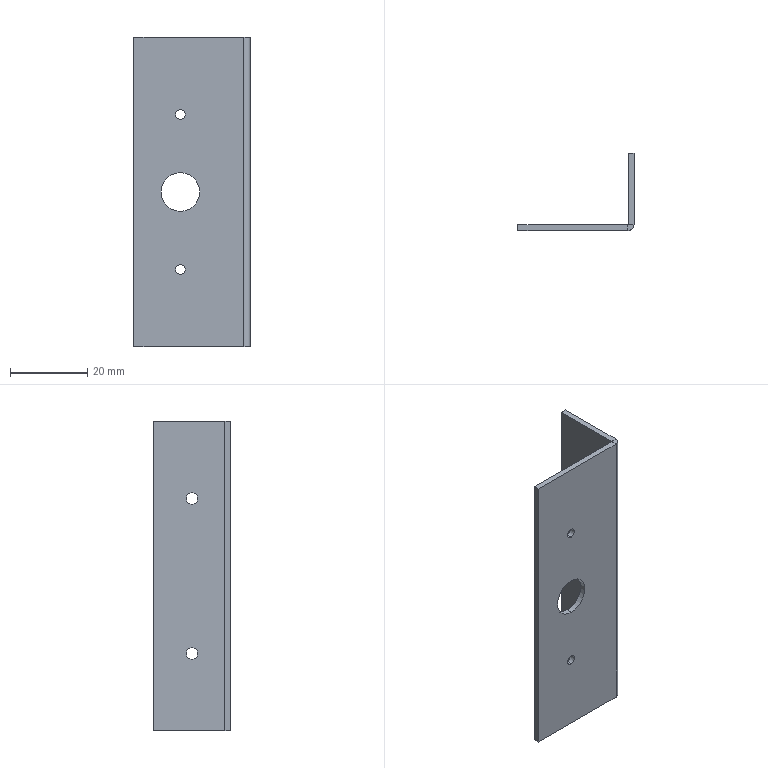Component | SolidWorks | LightBox-1_LampHolderMountingPlate-2 | 1 solid | 24 faces | box 30 x 20 x 80 mm | volume 5622 mm3 | cylinder 12 | plane 12 | commonest cylinder face diameters 3 x4 2.5 x4 10 x2 3.2 x1 0.2 x1
STEP:
#1=COLOUR_RGB('',0.7922,0.8196,0.9333);
#2=FILL_AREA_STYLE_COLOUR('',#1);
#3=FILL_AREA_STYLE('',(#2));
#4=SURFACE_STYLE_FILL_AREA(#3);
#5=SURFACE_SIDE_STYLE('',(#4));
#6=SURFACE_STYLE_USAGE(.BOTH.,#5);
#7=PRESENTATION_STYLE_ASSIGNMENT((#6));
#8=CARTESIAN_POINT('',(4.946,-0.2593,2.362));
#9=VERTEX_POINT('',#8);
#10=CARTESIAN_POINT('',(4.946,-0.1412,2.362));
#11=VERTEX_POINT('',#10);
#12=CARTESIAN_POINT('',(4.946,-0.2003,2.362));
#13=DIRECTION('',(1.,-0.,0.));
#14=DIRECTION('',(0.,1.,0.));
#15=AXIS2_PLACEMENT_3D('',#12,#13,#14);
#16=CIRCLE('',#15,0.05906);
#17=EDGE_CURVE('',#9,#11,#16,.T.);
#18=ORIENTED_EDGE('',*,*,#17,.F.);
#19=CARTESIAN_POINT('',(5.006,-0.2593,2.362));
#20=VERTEX_POINT('',#19);
#21=CARTESIAN_POINT('',(4.946,-0.2593,2.362));
#22=DIRECTION('',(1.,-0.,0.));
#23=VECTOR('',#22,39.37);
#24=LINE('',#21,#23);
#25=EDGE_CURVE('',#9,#20,#24,.T.);
#26=ORIENTED_EDGE('',*,*,#25,.T.);
#27=CARTESIAN_POINT('',(5.006,-0.1412,2.362));
#28=VERTEX_POINT('',#27);
#29=CARTESIAN_POINT('',(5.006,-0.2003,2.362));
#30=DIRECTION('',(1.,-0.,0.));
#31=DIRECTION('',(0.,1.,0.));
#32=AXIS2_PLACEMENT_3D('',#29,#30,#31);
#33=CIRCLE('',#32,0.05906);
#34=EDGE_CURVE('',#20,#28,#33,.T.);
#35=ORIENTED_EDGE('',*,*,#34,.T.);
#36=CARTESIAN_POINT('',(4.946,-0.1412,2.362));
#37=DIRECTION('',(1.,-0.,0.));
#38=VECTOR('',#37,39.37);
#39=LINE('',#36,#38);
#40=EDGE_CURVE('',#11,#28,#39,.T.);
#41=ORIENTED_EDGE('',*,*,#40,.F.);
#42=EDGE_LOOP('',(#18,#26,#35,#41));
#43=FACE_OUTER_BOUND('',#42,.T.);
#44=CARTESIAN_POINT('',(4.946,-0.2003,2.362));
#45=DIRECTION('',(1.,-0.,0.));
#46=DIRECTION('',(0.,1.,0.));
#47=AXIS2_PLACEMENT_3D('',#44,#45,#46);
#48=CYLINDRICAL_SURFACE('',#47,0.05906);
#49=ADVANCED_FACE('',(#43),#48,.F.);
#50=CARTESIAN_POINT('',(4.946,-0.2593,3.937));
#51=VERTEX_POINT('',#50);
#52=CARTESIAN_POINT('',(4.946,-0.1412,3.937));
#53=VERTEX_POINT('',#52);
#54=CARTESIAN_POINT('',(4.946,-0.2003,3.937));
#55=DIRECTION('',(1.,-0.,0.));
#56=DIRECTION('',(0.,1.,0.));
#57=AXIS2_PLACEMENT_3D('',#54,#55,#56);
#58=CIRCLE('',#57,0.05906);
#59=EDGE_CURVE('',#51,#53,#58,.T.);
#60=ORIENTED_EDGE('',*,*,#59,.F.);
#61=CARTESIAN_POINT('',(5.006,-0.2593,3.937));
#62=VERTEX_POINT('',#61);
#63=CARTESIAN_POINT('',(4.946,-0.2593,3.937));
#64=DIRECTION('',(1.,-0.,0.));
#65=VECTOR('',#64,39.37);
#66=LINE('',#63,#65);
#67=EDGE_CURVE('',#51,#62,#66,.T.);
#68=ORIENTED_EDGE('',*,*,#67,.T.);
#69=CARTESIAN_POINT('',(5.006,-0.1412,3.937));
#70=VERTEX_POINT('',#69);
#71=CARTESIAN_POINT('',(5.006,-0.2003,3.937));
#72=DIRECTION('',(1.,-0.,0.));
#73=DIRECTION('',(0.,1.,0.));
#74=AXIS2_PLACEMENT_3D('',#71,#72,#73);
#75=CIRCLE('',#74,0.05906);
#76=EDGE_CURVE('',#62,#70,#75,.T.);
#77=ORIENTED_EDGE('',*,*,#76,.T.);
#78=CARTESIAN_POINT('',(4.946,-0.1412,3.937));
#79=DIRECTION('',(1.,-0.,0.));
#80=VECTOR('',#79,39.37);
#81=LINE('',#78,#80);
#82=EDGE_CURVE('',#53,#70,#81,.T.);
#83=ORIENTED_EDGE('',*,*,#82,.F.);
#84=EDGE_LOOP('',(#60,#68,#77,#83));
#85=FACE_OUTER_BOUND('',#84,.T.);
#86=CARTESIAN_POINT('',(4.946,-0.2003,3.937));
#87=DIRECTION('',(1.,-0.,0.));
#88=DIRECTION('',(0.,1.,0.));
#89=AXIS2_PLACEMENT_3D('',#86,#87,#88);
#90=CYLINDRICAL_SURFACE('',#89,0.05906);
#91=ADVANCED_FACE('',(#85),#90,.F.);
#92=CARTESIAN_POINT('',(4.297,-0.594,2.313));
#93=VERTEX_POINT('',#92);
#94=CARTESIAN_POINT('',(4.297,-0.594,2.411));
#95=VERTEX_POINT('',#94);
#96=CARTESIAN_POINT('',(4.297,-0.594,2.362));
#97=DIRECTION('',(0.,1.,0.));
#98=DIRECTION('',(0.,0.,1.));
#99=AXIS2_PLACEMENT_3D('',#96,#97,#98);
#100=CIRCLE('',#99,0.04921);
#101=EDGE_CURVE('',#93,#95,#100,.T.);
#102=ORIENTED_EDGE('',*,*,#101,.F.);
#103=CARTESIAN_POINT('',(4.297,-0.5349,2.313));
#104=VERTEX_POINT('',#103);
#105=CARTESIAN_POINT('',(4.297,-0.594,2.313));
#106=DIRECTION('',(0.,1.,0.));
#107=VECTOR('',#106,39.37);
#108=LINE('',#105,#107);
#109=EDGE_CURVE('',#93,#104,#108,.T.);
#110=ORIENTED_EDGE('',*,*,#109,.T.);
#111=CARTESIAN_POINT('',(4.297,-0.5349,2.411));
#112=VERTEX_POINT('',#111);
#113=CARTESIAN_POINT('',(4.297,-0.5349,2.362));
#114=DIRECTION('',(0.,1.,0.));
#115=DIRECTION('',(0.,0.,1.));
#116=AXIS2_PLACEMENT_3D('',#113,#114,#115);
#117=CIRCLE('',#116,0.04921);
#118=EDGE_CURVE('',#104,#112,#117,.T.);
#119=ORIENTED_EDGE('',*,*,#118,.T.);
#120=CARTESIAN_POINT('',(4.297,-0.594,2.411));
#121=DIRECTION('',(0.,1.,0.));
#122=VECTOR('',#121,39.37);
#123=LINE('',#120,#122);
#124=EDGE_CURVE('',#95,#112,#123,.T.);
#125=ORIENTED_EDGE('',*,*,#124,.F.);
#126=EDGE_LOOP('',(#102,#110,#119,#125));
#127=FACE_OUTER_BOUND('',#126,.T.);
#128=CARTESIAN_POINT('',(4.297,-0.594,2.362));
#129=DIRECTION('',(0.,1.,0.));
#130=DIRECTION('',(0.,0.,1.));
#131=AXIS2_PLACEMENT_3D('',#128,#129,#130);
#132=CYLINDRICAL_SURFACE('',#131,0.04921);
#133=ADVANCED_FACE('',(#127),#132,.F.);
#134=CARTESIAN_POINT('',(4.297,-0.594,3.888));
#135=VERTEX_POINT('',#134);
#136=CARTESIAN_POINT('',(4.297,-0.594,3.986));
#137=VERTEX_POINT('',#136);
#138=CARTESIAN_POINT('',(4.297,-0.594,3.937));
#139=DIRECTION('',(0.,1.,0.));
#140=DIRECTION('',(0.,0.,1.));
#141=AXIS2_PLACEMENT_3D('',#138,#139,#140);
#142=CIRCLE('',#141,0.04921);
#143=EDGE_CURVE('',#135,#137,#142,.T.);
#144=ORIENTED_EDGE('',*,*,#143,.F.);
#145=CARTESIAN_POINT('',(4.297,-0.5349,3.888));
#146=VERTEX_POINT('',#145);
#147=CARTESIAN_POINT('',(4.297,-0.594,3.888));
#148=DIRECTION('',(0.,1.,0.));
#149=VECTOR('',#148,39.37);
#150=LINE('',#147,#149);
#151=EDGE_CURVE('',#135,#146,#150,.T.);
#152=ORIENTED_EDGE('',*,*,#151,.T.);
#153=CARTESIAN_POINT('',(4.297,-0.5349,3.986));
#154=VERTEX_POINT('',#153);
#155=CARTESIAN_POINT('',(4.297,-0.5349,3.937));
#156=DIRECTION('',(0.,1.,0.));
#157=DIRECTION('',(0.,0.,1.));
#158=AXIS2_PLACEMENT_3D('',#155,#156,#157);
#159=CIRCLE('',#158,0.04921);
#160=EDGE_CURVE('',#146,#154,#159,.T.);
#161=ORIENTED_EDGE('',*,*,#160,.T.);
#162=CARTESIAN_POINT('',(4.297,-0.594,3.986));
#163=DIRECTION('',(0.,1.,0.));
#164=VECTOR('',#163,39.37);
#165=LINE('',#162,#164);
#166=EDGE_CURVE('',#137,#154,#165,.T.);
#167=ORIENTED_EDGE('',*,*,#166,.F.);
#168=EDGE_LOOP('',(#144,#152,#161,#167));
#169=FACE_OUTER_BOUND('',#168,.T.);
#170=CARTESIAN_POINT('',(4.297,-0.594,3.937));
#171=DIRECTION('',(0.,1.,0.));
#172=DIRECTION('',(0.,0.,1.));
#173=AXIS2_PLACEMENT_3D('',#170,#171,#172);
#174=CYLINDRICAL_SURFACE('',#173,0.04921);
#175=ADVANCED_FACE('',(#169),#174,.F.);
#176=CARTESIAN_POINT('',(4.297,-0.594,2.953));
#177=VERTEX_POINT('',#176);
#178=CARTESIAN_POINT('',(4.297,-0.594,3.346));
#179=VERTEX_POINT('',#178);
#180=CARTESIAN_POINT('',(4.297,-0.594,3.15));
#181=DIRECTION('',(0.,1.,0.));
#182=DIRECTION('',(0.,0.,1.));
#183=AXIS2_PLACEMENT_3D('',#180,#181,#182);
#184=CIRCLE('',#183,0.1969);
#185=EDGE_CURVE('',#177,#179,#184,.T.);
#186=ORIENTED_EDGE('',*,*,#185,.F.);
#187=CARTESIAN_POINT('',(4.297,-0.5349,2.953));
#188=VERTEX_POINT('',#187);
#189=CARTESIAN_POINT('',(4.297,-0.594,2.953));
#190=DIRECTION('',(0.,1.,0.));
#191=VECTOR('',#190,39.37);
#192=LINE('',#189,#191);
#193=EDGE_CURVE('',#177,#188,#192,.T.);
#194=ORIENTED_EDGE('',*,*,#193,.T.);
#195=CARTESIAN_POINT('',(4.297,-0.5349,3.346));
#196=VERTEX_POINT('',#195);
#197=CARTESIAN_POINT('',(4.297,-0.5349,3.15));
#198=DIRECTION('',(0.,1.,0.));
#199=DIRECTION('',(0.,0.,1.));
#200=AXIS2_PLACEMENT_3D('',#197,#198,#199);
#201=CIRCLE('',#200,0.1969);
#202=EDGE_CURVE('',#188,#196,#201,.T.);
#203=ORIENTED_EDGE('',*,*,#202,.T.);
#204=CARTESIAN_POINT('',(4.297,-0.594,3.346));
#205=DIRECTION('',(0.,1.,0.));
#206=VECTOR('',#205,39.37);
#207=LINE('',#204,#206);
#208=EDGE_CURVE('',#179,#196,#207,.T.);
#209=ORIENTED_EDGE('',*,*,#208,.F.);
#210=EDGE_LOOP('',(#186,#194,#203,#209));
#211=FACE_OUTER_BOUND('',#210,.T.);
#212=CARTESIAN_POINT('',(4.297,-0.594,3.15));
#213=DIRECTION('',(0.,1.,0.));
#214=DIRECTION('',(0.,0.,1.));
#215=AXIS2_PLACEMENT_3D('',#212,#213,#214);
#216=CYLINDRICAL_SURFACE('',#215,0.1969);
#217=ADVANCED_FACE('',(#211),#216,.F.);
#218=CARTESIAN_POINT('',(4.943,-0.5349,1.575));
#219=VERTEX_POINT('',#218);
#220=CARTESIAN_POINT('',(3.824,-0.5349,1.575));
#221=VERTEX_POINT('',#220);
#222=CARTESIAN_POINT('',(3.824,-0.5349,1.575));
#223=DIRECTION('',(-1.,0.,0.));
#224=VECTOR('',#223,39.37);
#225=LINE('',#222,#224);
#226=EDGE_CURVE('',#219,#221,#225,.T.);
#227=ORIENTED_EDGE('',*,*,#226,.F.);
#228=CARTESIAN_POINT('',(4.943,-0.594,1.575));
#229=VERTEX_POINT('',#228);
#230=CARTESIAN_POINT('',(4.943,-0.5349,1.575));
#231=DIRECTION('',(0.,-1.,0.));
#232=VECTOR('',#231,39.37);
#233=LINE('',#230,#232);
#234=EDGE_CURVE('',#219,#229,#233,.T.);
#235=ORIENTED_EDGE('',*,*,#234,.T.);
#236=CARTESIAN_POINT('',(3.824,-0.594,1.575));
#237=VERTEX_POINT('',#236);
#238=CARTESIAN_POINT('',(3.824,-0.594,1.575));
#239=DIRECTION('',(-1.,0.,0.));
#240=VECTOR('',#239,39.37);
#241=LINE('',#238,#240);
#242=EDGE_CURVE('',#229,#237,#241,.T.);
#243=ORIENTED_EDGE('',*,*,#242,.T.);
#244=CARTESIAN_POINT('',(3.824,-0.594,1.575));
#245=DIRECTION('',(0.,1.,0.));
#246=VECTOR('',#245,39.37);
#247=LINE('',#244,#246);
#248=EDGE_CURVE('',#237,#221,#247,.T.);
#249=ORIENTED_EDGE('',*,*,#248,.T.);
#250=EDGE_LOOP('',(#227,#235,#243,#249));
#251=FACE_OUTER_BOUND('',#250,.T.);
#252=CARTESIAN_POINT('',(3.824,-0.594,1.575));
#253=DIRECTION('',(0.,0.,-1.));
#254=DIRECTION('',(-1.,0.,0.));
#255=AXIS2_PLACEMENT_3D('',#252,#253,#254);
#256=PLANE('',#255);
#257=ADVANCED_FACE('',(#251),#256,.T.);
#258=CARTESIAN_POINT('',(4.297,-0.594,2.362));
#259=DIRECTION('',(0.,1.,0.));
#260=DIRECTION('',(0.,0.,1.));
#261=AXIS2_PLACEMENT_3D('',#258,#259,#260);
#262=CIRCLE('',#261,0.04921);
#263=EDGE_CURVE('',#95,#93,#262,.T.);
#264=ORIENTED_EDGE('',*,*,#263,.T.);
#265=ORIENTED_EDGE('',*,*,#101,.T.);
#266=EDGE_LOOP('',(#264,#265));
#267=FACE_BOUND('',#266,.T.);
#268=CARTESIAN_POINT('',(4.297,-0.594,3.937));
#269=DIRECTION('',(0.,1.,0.));
#270=DIRECTION('',(0.,0.,1.));
#271=AXIS2_PLACEMENT_3D('',#268,#269,#270);
#272=CIRCLE('',#271,0.04921);
#273=EDGE_CURVE('',#137,#135,#272,.T.);
#274=ORIENTED_EDGE('',*,*,#273,.T.);
#275=ORIENTED_EDGE('',*,*,#143,.T.);
#276=EDGE_LOOP('',(#274,#275));
#277=FACE_BOUND('',#276,.T.);
#278=CARTESIAN_POINT('',(4.297,-0.594,3.15));
#279=DIRECTION('',(0.,1.,0.));
#280=DIRECTION('',(0.,0.,1.));
#281=AXIS2_PLACEMENT_3D('',#278,#279,#280);
#282=CIRCLE('',#281,0.1969);
#283=EDGE_CURVE('',#179,#177,#282,.T.);
#284=ORIENTED_EDGE('',*,*,#283,.T.);
#285=ORIENTED_EDGE('',*,*,#185,.T.);
#286=EDGE_LOOP('',(#284,#285));
#287=FACE_BOUND('',#286,.T.);
#288=ORIENTED_EDGE('',*,*,#242,.F.);
#289=CARTESIAN_POINT('',(4.943,-0.594,4.724));
#290=VERTEX_POINT('',#289);
#291=CARTESIAN_POINT('',(4.943,-0.594,1.575));
#292=DIRECTION('',(0.,0.,1.));
#293=VECTOR('',#292,39.37);
#294=LINE('',#291,#293);
#295=EDGE_CURVE('',#229,#290,#294,.T.);
#296=ORIENTED_EDGE('',*,*,#295,.T.);
#297=CARTESIAN_POINT('',(3.824,-0.594,4.724));
#298=VERTEX_POINT('',#297);
#299=CARTESIAN_POINT('',(3.824,-0.594,4.724));
#300=DIRECTION('',(1.,0.,0.));
#301=VECTOR('',#300,39.37);
#302=LINE('',#299,#301);
#303=EDGE_CURVE('',#298,#290,#302,.T.);
#304=ORIENTED_EDGE('',*,*,#303,.F.);
#305=CARTESIAN_POINT('',(3.824,-0.594,4.724));
#306=DIRECTION('',(0.,0.,1.));
#307=VECTOR('',#306,39.37);
#308=LINE('',#305,#307);
#309=EDGE_CURVE('',#237,#298,#308,.T.);
#310=ORIENTED_EDGE('',*,*,#309,.F.);
#311=EDGE_LOOP('',(#288,#296,#304,#310));
#312=FACE_OUTER_BOUND('',#311,.T.);
#313=CARTESIAN_POINT('',(6.267,-0.594,3.173));
#314=DIRECTION('',(0.,-1.,0.));
#315=DIRECTION('',(0.,0.,-1.));
#316=AXIS2_PLACEMENT_3D('',#313,#314,#315);
#317=PLANE('',#316);
#318=ADVANCED_FACE('',(#267,#277,#287,#312),#317,.T.);
#319=CARTESIAN_POINT('',(4.297,-0.5349,3.15));
#320=DIRECTION('',(0.,1.,0.));
#321=DIRECTION('',(0.,0.,1.));
#322=AXIS2_PLACEMENT_3D('',#319,#320,#321);
#323=CIRCLE('',#322,0.1969);
#324=EDGE_CURVE('',#196,#188,#323,.T.);
#325=ORIENTED_EDGE('',*,*,#324,.F.);
#326=ORIENTED_EDGE('',*,*,#202,.F.);
#327=EDGE_LOOP('',(#325,#326));
#328=FACE_BOUND('',#327,.T.);
#329=CARTESIAN_POINT('',(4.297,-0.5349,3.937));
#330=DIRECTION('',(0.,1.,0.));
#331=DIRECTION('',(0.,0.,1.));
#332=AXIS2_PLACEMENT_3D('',#329,#330,#331);
#333=CIRCLE('',#332,0.04921);
#334=EDGE_CURVE('',#154,#146,#333,.T.);
#335=ORIENTED_EDGE('',*,*,#334,.F.);
#336=ORIENTED_EDGE('',*,*,#160,.F.);
#337=EDGE_LOOP('',(#335,#336));
#338=FACE_BOUND('',#337,.T.);
#339=CARTESIAN_POINT('',(4.297,-0.5349,2.362));
#340=DIRECTION('',(0.,1.,0.));
#341=DIRECTION('',(0.,0.,1.));
#342=AXIS2_PLACEMENT_3D('',#339,#340,#341);
#343=CIRCLE('',#342,0.04921);
#344=EDGE_CURVE('',#112,#104,#343,.T.);
#345=ORIENTED_EDGE('',*,*,#344,.F.);
#346=ORIENTED_EDGE('',*,*,#118,.F.);
#347=EDGE_LOOP('',(#345,#346));
#348=FACE_BOUND('',#347,.T.);
#349=CARTESIAN_POINT('',(4.943,-0.5349,4.724));
#350=VERTEX_POINT('',#349);
#351=CARTESIAN_POINT('',(4.943,-0.5349,1.575));
#352=DIRECTION('',(0.,0.,1.));
#353=VECTOR('',#352,39.37);
#354=LINE('',#351,#353);
#355=EDGE_CURVE('',#219,#350,#354,.T.);
#356=ORIENTED_EDGE('',*,*,#355,.F.);
#357=ORIENTED_EDGE('',*,*,#226,.T.);
#358=CARTESIAN_POINT('',(3.824,-0.5349,4.724));
#359=VERTEX_POINT('',#358);
#360=CARTESIAN_POINT('',(3.824,-0.5349,4.724));
#361=DIRECTION('',(0.,0.,1.));
#362=VECTOR('',#361,39.37);
#363=LINE('',#360,#362);
#364=EDGE_CURVE('',#221,#359,#363,.T.);
#365=ORIENTED_EDGE('',*,*,#364,.T.);
#366=CARTESIAN_POINT('',(3.824,-0.5349,4.724));
#367=DIRECTION('',(1.,0.,0.));
#368=VECTOR('',#367,39.37);
#369=LINE('',#366,#368);
#370=EDGE_CURVE('',#359,#350,#369,.T.);
#371=ORIENTED_EDGE('',*,*,#370,.T.);
#372=EDGE_LOOP('',(#356,#357,#365,#371));
#373=FACE_OUTER_BOUND('',#372,.T.);
#374=CARTESIAN_POINT('',(6.267,-0.5349,3.173));
#375=DIRECTION('',(0.,-1.,0.));
#376=DIRECTION('',(0.,0.,-1.));
#377=AXIS2_PLACEMENT_3D('',#374,#375,#376);
#378=PLANE('',#377);
#379=ADVANCED_FACE('',(#328,#338,#348,#373),#378,.F.);
#380=ORIENTED_EDGE('',*,*,#364,.F.);
#381=ORIENTED_EDGE('',*,*,#248,.F.);
#382=ORIENTED_EDGE('',*,*,#309,.T.);
#383=CARTESIAN_POINT('',(3.824,-0.594,4.724));
#384=DIRECTION('',(0.,1.,0.));
#385=VECTOR('',#384,39.37);
#386=LINE('',#383,#385);
#387=EDGE_CURVE('',#298,#359,#386,.T.);
#388=ORIENTED_EDGE('',*,*,#387,.T.);
#389=EDGE_LOOP('',(#380,#381,#382,#388));
#390=FACE_OUTER_BOUND('',#389,.T.);
#391=CARTESIAN_POINT('',(3.824,-0.594,4.724));
#392=DIRECTION('',(-1.,0.,0.));
#393=DIRECTION('',(0.,0.,1.));
#394=AXIS2_PLACEMENT_3D('',#391,#392,#393);
#395=PLANE('',#394);
#396=ADVANCED_FACE('',(#390),#395,.T.);
#397=CARTESIAN_POINT('',(4.943,-0.5349,4.724));
#398=DIRECTION('',(0.,-1.,0.));
#399=VECTOR('',#398,39.37);
#400=LINE('',#397,#399);
#401=EDGE_CURVE('',#350,#290,#400,.T.);
#402=ORIENTED_EDGE('',*,*,#401,.F.);
#403=ORIENTED_EDGE('',*,*,#370,.F.);
#404=ORIENTED_EDGE('',*,*,#387,.F.);
#405=ORIENTED_EDGE('',*,*,#303,.T.);
#406=EDGE_LOOP('',(#402,#403,#404,#405));
#407=FACE_OUTER_BOUND('',#406,.T.);
#408=CARTESIAN_POINT('',(3.824,-0.594,4.724));
#409=DIRECTION('',(0.,0.,1.));
#410=DIRECTION('',(1.,0.,0.));
#411=AXIS2_PLACEMENT_3D('',#408,#409,#410);
#412=PLANE('',#411);
#413=ADVANCED_FACE('',(#407),#412,.T.);
#414=ORIENTED_EDGE('',*,*,#193,.F.);
#415=ORIENTED_EDGE('',*,*,#283,.F.);
#416=ORIENTED_EDGE('',*,*,#208,.T.);
#417=ORIENTED_EDGE('',*,*,#324,.T.);
#418=EDGE_LOOP('',(#414,#415,#416,#417));
#419=FACE_OUTER_BOUND('',#418,.T.);
#420=CARTESIAN_POINT('',(4.297,-0.594,3.15));
#421=DIRECTION('',(0.,1.,0.));
#422=DIRECTION('',(0.,0.,1.));
#423=AXIS2_PLACEMENT_3D('',#420,#421,#422);
#424=CYLINDRICAL_SURFACE('',#423,0.1969);
#425=ADVANCED_FACE('',(#419),#424,.F.);
#426=ORIENTED_EDGE('',*,*,#151,.F.);
#427=ORIENTED_EDGE('',*,*,#273,.F.);
#428=ORIENTED_EDGE('',*,*,#166,.T.);
#429=ORIENTED_EDGE('',*,*,#334,.T.);
#430=EDGE_LOOP('',(#426,#427,#428,#429));
#431=FACE_OUTER_BOUND('',#430,.T.);
#432=CARTESIAN_POINT('',(4.297,-0.594,3.937));
#433=DIRECTION('',(0.,1.,0.));
#434=DIRECTION('',(0.,0.,1.));
#435=AXIS2_PLACEMENT_3D('',#432,#433,#434);
#436=CYLINDRICAL_SURFACE('',#435,0.04921);
#437=ADVANCED_FACE('',(#431),#436,.F.);
#438=ORIENTED_EDGE('',*,*,#109,.F.);
#439=ORIENTED_EDGE('',*,*,#263,.F.);
#440=ORIENTED_EDGE('',*,*,#124,.T.);
#441=ORIENTED_EDGE('',*,*,#344,.T.);
#442=EDGE_LOOP('',(#438,#439,#440,#441));
#443=FACE_OUTER_BOUND('',#442,.T.);
#444=CARTESIAN_POINT('',(4.297,-0.594,2.362));
#445=DIRECTION('',(0.,1.,0.));
#446=DIRECTION('',(0.,0.,1.));
#447=AXIS2_PLACEMENT_3D('',#444,#445,#446);
#448=CYLINDRICAL_SURFACE('',#447,0.04921);
#449=ADVANCED_FACE('',(#443),#448,.F.);
#450=CARTESIAN_POINT('',(4.946,-0.531,4.724));
#451=VERTEX_POINT('',#450);
#452=CARTESIAN_POINT('',(5.006,-0.531,4.724));
#453=VERTEX_POINT('',#452);
#454=CARTESIAN_POINT('',(5.006,-0.531,4.724));
#455=DIRECTION('',(1.,-0.,0.));
#456=VECTOR('',#455,39.37);
#457=LINE('',#454,#456);
#458=EDGE_CURVE('',#451,#453,#457,.T.);
#459=ORIENTED_EDGE('',*,*,#458,.F.);
#460=CARTESIAN_POINT('',(4.943,-0.531,4.724));
#461=DIRECTION('',(0.,0.,1.));
#462=DIRECTION('',(-1.,0.,0.));
#463=AXIS2_PLACEMENT_3D('',#460,#461,#462);
#464=CIRCLE('',#463,0.003937);
#465=EDGE_CURVE('',#350,#451,#464,.T.);
#466=ORIENTED_EDGE('',*,*,#465,.F.);
#467=ORIENTED_EDGE('',*,*,#401,.T.);
#468=CARTESIAN_POINT('',(4.943,-0.531,4.724));
#469=DIRECTION('',(0.,0.,1.));
#470=DIRECTION('',(-1.,0.,0.));
#471=AXIS2_PLACEMENT_3D('',#468,#469,#470);
#472=CIRCLE('',#471,0.06299);
#473=EDGE_CURVE('',#290,#453,#472,.T.);
#474=ORIENTED_EDGE('',*,*,#473,.T.);
#475=EDGE_LOOP('',(#459,#466,#467,#474));
#476=FACE_OUTER_BOUND('',#475,.T.);
#477=CARTESIAN_POINT('',(4.943,-0.531,4.724));
#478=DIRECTION('',(0.,0.,1.));
#479=DIRECTION('',(1.,0.,0.));
#480=AXIS2_PLACEMENT_3D('',#477,#478,#479);
#481=PLANE('',#480);
#482=ADVANCED_FACE('',(#476),#481,.T.);
#483=CARTESIAN_POINT('',(4.946,-0.531,1.575));
#484=VERTEX_POINT('',#483);
#485=CARTESIAN_POINT('',(4.943,-0.531,1.575));
#486=DIRECTION('',(0.,0.,-1.));
#487=DIRECTION('',(-1.,0.,0.));
#488=AXIS2_PLACEMENT_3D('',#485,#486,#487);
#489=CIRCLE('',#488,0.003937);
#490=EDGE_CURVE('',#484,#219,#489,.T.);
#491=ORIENTED_EDGE('',*,*,#490,.F.);
#492=CARTESIAN_POINT('',(5.006,-0.531,1.575));
#493=VERTEX_POINT('',#492);
#494=CARTESIAN_POINT('',(4.946,-0.531,1.575));
#495=DIRECTION('',(1.,-0.,0.));
#496=VECTOR('',#495,39.37);
#497=LINE('',#494,#496);
#498=EDGE_CURVE('',#484,#493,#497,.T.);
#499=ORIENTED_EDGE('',*,*,#498,.T.);
#500=CARTESIAN_POINT('',(4.943,-0.531,1.575));
#501=DIRECTION('',(0.,0.,-1.));
#502=DIRECTION('',(-1.,0.,0.));
#503=AXIS2_PLACEMENT_3D('',#500,#501,#502);
#504=CIRCLE('',#503,0.06299);
#505=EDGE_CURVE('',#493,#229,#504,.T.);
#506=ORIENTED_EDGE('',*,*,#505,.T.);
#507=ORIENTED_EDGE('',*,*,#234,.F.);
#508=EDGE_LOOP('',(#491,#499,#506,#507));
#509=FACE_OUTER_BOUND('',#508,.T.);
#510=CARTESIAN_POINT('',(4.943,-0.531,1.575));
#511=DIRECTION('',(0.,0.,1.));
#512=DIRECTION('',(1.,0.,0.));
#513=AXIS2_PLACEMENT_3D('',#510,#511,#512);
#514=PLANE('',#513);
#515=ADVANCED_FACE('',(#509),#514,.F.);
#516=ORIENTED_EDGE('',*,*,#295,.F.);
#517=ORIENTED_EDGE('',*,*,#505,.F.);
#518=CARTESIAN_POINT('',(5.006,-0.531,3.173));
#519=DIRECTION('',(0.,0.,-1.));
#520=VECTOR('',#519,39.37);
#521=LINE('',#518,#520);
#522=EDGE_CURVE('',#453,#493,#521,.T.);
#523=ORIENTED_EDGE('',*,*,#522,.F.);
#524=ORIENTED_EDGE('',*,*,#473,.F.);
#525=EDGE_LOOP('',(#516,#517,#523,#524));
#526=FACE_OUTER_BOUND('',#525,.T.);
#527=CARTESIAN_POINT('',(4.943,-0.531,1.575));
#528=DIRECTION('',(0.,0.,-1.));
#529=DIRECTION('',(1.,-0.,0.));
#530=AXIS2_PLACEMENT_3D('',#527,#528,#529);
#531=CYLINDRICAL_SURFACE('',#530,0.06299);
#532=ADVANCED_FACE('',(#526),#531,.T.);
#533=ORIENTED_EDGE('',*,*,#355,.T.);
#534=ORIENTED_EDGE('',*,*,#465,.T.);
#535=CARTESIAN_POINT('',(4.946,-0.531,4.724));
#536=DIRECTION('',(0.,0.,-1.));
#537=VECTOR('',#536,39.37);
#538=LINE('',#535,#537);
#539=EDGE_CURVE('',#451,#484,#538,.T.);
#540=ORIENTED_EDGE('',*,*,#539,.T.);
#541=ORIENTED_EDGE('',*,*,#490,.T.);
#542=EDGE_LOOP('',(#533,#534,#540,#541));
#543=FACE_OUTER_BOUND('',#542,.T.);
#544=CARTESIAN_POINT('',(4.943,-0.531,1.575));
#545=DIRECTION('',(0.,0.,-1.));
#546=DIRECTION('',(1.,0.,0.));
#547=AXIS2_PLACEMENT_3D('',#544,#545,#546);
#548=CYLINDRICAL_SURFACE('',#547,0.003937);
#549=ADVANCED_FACE('',(#543),#548,.F.);
#550=CARTESIAN_POINT('',(5.006,0.1934,1.575));
#551=VERTEX_POINT('',#550);
#552=CARTESIAN_POINT('',(5.006,-0.5349,1.575));
#553=DIRECTION('',(-0.,-1.,0.));
#554=VECTOR('',#553,39.37);
#555=LINE('',#552,#554);
#556=EDGE_CURVE('',#551,#493,#555,.T.);
#557=ORIENTED_EDGE('',*,*,#556,.T.);
#558=ORIENTED_EDGE('',*,*,#498,.F.);
#559=CARTESIAN_POINT('',(4.946,0.1934,1.575));
#560=VERTEX_POINT('',#559);
#561=CARTESIAN_POINT('',(4.946,-0.5349,1.575));
#562=DIRECTION('',(-0.,-1.,0.));
#563=VECTOR('',#562,39.37);
#564=LINE('',#561,#563);
#565=EDGE_CURVE('',#560,#484,#564,.T.);
#566=ORIENTED_EDGE('',*,*,#565,.F.);
#567=CARTESIAN_POINT('',(5.006,0.1934,1.575));
#568=DIRECTION('',(-1.,0.,0.));
#569=VECTOR('',#568,39.37);
#570=LINE('',#567,#569);
#571=EDGE_CURVE('',#551,#560,#570,.T.);
#572=ORIENTED_EDGE('',*,*,#571,.F.);
#573=EDGE_LOOP('',(#557,#558,#566,#572));
#574=FACE_OUTER_BOUND('',#573,.T.);
#575=CARTESIAN_POINT('',(5.006,-0.5349,1.575));
#576=DIRECTION('',(0.,0.,-1.));
#577=DIRECTION('',(-1.,0.,0.));
#578=AXIS2_PLACEMENT_3D('',#575,#576,#577);
#579=PLANE('',#578);
#580=ADVANCED_FACE('',(#574),#579,.T.);
#581=CARTESIAN_POINT('',(4.946,0.1934,4.724));
#582=VERTEX_POINT('',#581);
#583=CARTESIAN_POINT('',(4.946,-0.5349,4.724));
#584=DIRECTION('',(0.,1.,0.));
#585=VECTOR('',#584,39.37);
#586=LINE('',#583,#585);
#587=EDGE_CURVE('',#451,#582,#586,.T.);
#588=ORIENTED_EDGE('',*,*,#587,.F.);
#589=ORIENTED_EDGE('',*,*,#458,.T.);
#590=CARTESIAN_POINT('',(5.006,0.1934,4.724));
#591=VERTEX_POINT('',#590);
#592=CARTESIAN_POINT('',(5.006,0.1934,4.724));
#593=DIRECTION('',(0.,1.,0.));
#594=VECTOR('',#593,39.37);
#595=LINE('',#592,#594);
#596=EDGE_CURVE('',#453,#591,#595,.T.);
#597=ORIENTED_EDGE('',*,*,#596,.T.);
#598=CARTESIAN_POINT('',(5.006,0.1934,4.724));
#599=DIRECTION('',(-1.,0.,0.));
#600=VECTOR('',#599,39.37);
#601=LINE('',#598,#600);
#602=EDGE_CURVE('',#591,#582,#601,.T.);
#603=ORIENTED_EDGE('',*,*,#602,.T.);
#604=EDGE_LOOP('',(#588,#589,#597,#603));
#605=FACE_OUTER_BOUND('',#604,.T.);
#606=CARTESIAN_POINT('',(5.006,0.1934,4.724));
#607=DIRECTION('',(0.,0.,1.));
#608=DIRECTION('',(1.,0.,0.));
#609=AXIS2_PLACEMENT_3D('',#606,#607,#608);
#610=PLANE('',#609);
#611=ADVANCED_FACE('',(#605),#610,.T.);
#612=CARTESIAN_POINT('',(5.006,-0.2003,2.362));
#613=DIRECTION('',(1.,-0.,0.));
#614=DIRECTION('',(0.,1.,0.));
#615=AXIS2_PLACEMENT_3D('',#612,#613,#614);
#616=CIRCLE('',#615,0.05906);
#617=EDGE_CURVE('',#28,#20,#616,.T.);
#618=ORIENTED_EDGE('',*,*,#617,.F.);
#619=ORIENTED_EDGE('',*,*,#34,.F.);
#620=EDGE_LOOP('',(#618,#619));
#621=FACE_BOUND('',#620,.T.);
#622=CARTESIAN_POINT('',(5.006,-0.2003,3.937));
#623=DIRECTION('',(1.,-0.,0.));
#624=DIRECTION('',(0.,1.,0.));
#625=AXIS2_PLACEMENT_3D('',#622,#623,#624);
#626=CIRCLE('',#625,0.05906);
#627=EDGE_CURVE('',#70,#62,#626,.T.);
#628=ORIENTED_EDGE('',*,*,#627,.F.);
#629=ORIENTED_EDGE('',*,*,#76,.F.);
#630=EDGE_LOOP('',(#628,#629));
#631=FACE_BOUND('',#630,.T.);
#632=ORIENTED_EDGE('',*,*,#596,.F.);
#633=ORIENTED_EDGE('',*,*,#522,.T.);
#634=ORIENTED_EDGE('',*,*,#556,.F.);
#635=CARTESIAN_POINT('',(5.006,0.1934,1.575));
#636=DIRECTION('',(0.,0.,-1.));
#637=VECTOR('',#636,39.37);
#638=LINE('',#635,#637);
#639=EDGE_CURVE('',#591,#551,#638,.T.);
#640=ORIENTED_EDGE('',*,*,#639,.F.);
#641=EDGE_LOOP('',(#632,#633,#634,#640));
#642=FACE_OUTER_BOUND('',#641,.T.);
#643=CARTESIAN_POINT('',(5.006,-0.5349,3.173));
#644=DIRECTION('',(1.,-0.,0.));
#645=DIRECTION('',(0.,1.,0.));
#646=AXIS2_PLACEMENT_3D('',#643,#644,#645);
#647=PLANE('',#646);
#648=ADVANCED_FACE('',(#621,#631,#642),#647,.T.);
#649=CARTESIAN_POINT('',(4.946,-0.2003,2.362));
#650=DIRECTION('',(1.,-0.,0.));
#651=DIRECTION('',(0.,1.,0.));
#652=AXIS2_PLACEMENT_3D('',#649,#650,#651);
#653=CIRCLE('',#652,0.05906);
#654=EDGE_CURVE('',#11,#9,#653,.T.);
#655=ORIENTED_EDGE('',*,*,#654,.T.);
#656=ORIENTED_EDGE('',*,*,#17,.T.);
#657=EDGE_LOOP('',(#655,#656));
#658=FACE_BOUND('',#657,.T.);
#659=CARTESIAN_POINT('',(4.946,-0.2003,3.937));
#660=DIRECTION('',(1.,-0.,0.));
#661=DIRECTION('',(0.,1.,0.));
#662=AXIS2_PLACEMENT_3D('',#659,#660,#661);
#663=CIRCLE('',#662,0.05906);
#664=EDGE_CURVE('',#53,#51,#663,.T.);
#665=ORIENTED_EDGE('',*,*,#664,.T.);
#666=ORIENTED_EDGE('',*,*,#59,.T.);
#667=EDGE_LOOP('',(#665,#666));
#668=FACE_BOUND('',#667,.T.);
#669=ORIENTED_EDGE('',*,*,#539,.F.);
#670=ORIENTED_EDGE('',*,*,#587,.T.);
#671=CARTESIAN_POINT('',(4.946,0.1934,3.173));
#672=DIRECTION('',(0.,0.,-1.));
#673=VECTOR('',#672,39.37);
#674=LINE('',#671,#673);
#675=EDGE_CURVE('',#582,#560,#674,.T.);
#676=ORIENTED_EDGE('',*,*,#675,.T.);
#677=ORIENTED_EDGE('',*,*,#565,.T.);
#678=EDGE_LOOP('',(#669,#670,#676,#677));
#679=FACE_OUTER_BOUND('',#678,.T.);
#680=CARTESIAN_POINT('',(4.946,-0.5349,3.173));
#681=DIRECTION('',(1.,-0.,0.));
#682=DIRECTION('',(0.,1.,0.));
#683=AXIS2_PLACEMENT_3D('',#680,#681,#682);
#684=PLANE('',#683);
#685=ADVANCED_FACE('',(#658,#668,#679),#684,.F.);
#686=ORIENTED_EDGE('',*,*,#675,.F.);
#687=ORIENTED_EDGE('',*,*,#602,.F.);
#688=ORIENTED_EDGE('',*,*,#639,.T.);
#689=ORIENTED_EDGE('',*,*,#571,.T.);
#690=EDGE_LOOP('',(#686,#687,#688,#689));
#691=FACE_OUTER_BOUND('',#690,.T.);
#692=CARTESIAN_POINT('',(5.006,0.1934,1.575));
#693=DIRECTION('',(0.,1.,0.));
#694=DIRECTION('',(-1.,0.,0.));
#695=AXIS2_PLACEMENT_3D('',#692,#693,#694);
#696=PLANE('',#695);
#697=ADVANCED_FACE('',(#691),#696,.T.);
#698=ORIENTED_EDGE('',*,*,#67,.F.);
#699=ORIENTED_EDGE('',*,*,#664,.F.);
#700=ORIENTED_EDGE('',*,*,#82,.T.);
#701=ORIENTED_EDGE('',*,*,#627,.T.);
#702=EDGE_LOOP('',(#698,#699,#700,#701));
#703=FACE_OUTER_BOUND('',#702,.T.);
#704=CARTESIAN_POINT('',(4.946,-0.2003,3.937));
#705=DIRECTION('',(1.,-0.,0.));
#706=DIRECTION('',(0.,1.,0.));
#707=AXIS2_PLACEMENT_3D('',#704,#705,#706);
#708=CYLINDRICAL_SURFACE('',#707,0.05906);
#709=ADVANCED_FACE('',(#703),#708,.F.);
#710=ORIENTED_EDGE('',*,*,#25,.F.);
#711=ORIENTED_EDGE('',*,*,#654,.F.);
#712=ORIENTED_EDGE('',*,*,#40,.T.);
#713=ORIENTED_EDGE('',*,*,#617,.T.);
#714=EDGE_LOOP('',(#710,#711,#712,#713));
#715=FACE_OUTER_BOUND('',#714,.T.);
#716=CARTESIAN_POINT('',(4.946,-0.2003,2.362));
#717=DIRECTION('',(1.,-0.,0.));
#718=DIRECTION('',(0.,1.,0.));
#719=AXIS2_PLACEMENT_3D('',#716,#717,#718);
#720=CYLINDRICAL_SURFACE('',#719,0.05906);
#721=ADVANCED_FACE('',(#715),#720,.F.);
#722=CLOSED_SHELL('',(#49,#91,#133,#175,#217,#257,#318,#379,#396,#413,#425,#437,#449,#482,#515,#532,#549,#580,#611,#648,#685,#697,#709,#721));
#723=MANIFOLD_SOLID_BREP('',#722);
#724=STYLED_ITEM('',(#7),#723);
#725=PRESENTATION_LAYER_ASSIGNMENT('','',(#724));
#726=(LENGTH_UNIT()NAMED_UNIT(*)SI_UNIT($,.METRE.));
#727=LENGTH_MEASURE_WITH_UNIT(LENGTH_MEASURE(0.0254),#726);
#728=DIMENSIONAL_EXPONENTS(1.,0.,0.,0.,0.,0.,0.);
#729=(CONVERSION_BASED_UNIT('',#727)LENGTH_UNIT()NAMED_UNIT(#728));
#730=UNCERTAINTY_MEASURE_WITH_UNIT(LENGTH_MEASURE(0.00001),#729,'','');
#731=(NAMED_UNIT(*)PLANE_ANGLE_UNIT()SI_UNIT($,.RADIAN.));
#732=(NAMED_UNIT(*)SI_UNIT($,.STERADIAN.)SOLID_ANGLE_UNIT());
#733=(GEOMETRIC_REPRESENTATION_CONTEXT(3)GLOBAL_UNCERTAINTY_ASSIGNED_CONTEXT((#730))GLOBAL_UNIT_ASSIGNED_CONTEXT((#729,#731,#732))REPRESENTATION_CONTEXT('',''));
#734=MECHANICAL_DESIGN_GEOMETRIC_PRESENTATION_REPRESENTATION('',(#724),#733);
#735=CARTESIAN_POINT('',(0.,0.,0.));
#736=DIRECTION('',(0.,0.,1.));
#737=DIRECTION('',(1.,0.,0.));
#738=AXIS2_PLACEMENT_3D('',#735,#736,#737);
#739=(LENGTH_UNIT()NAMED_UNIT(*)SI_UNIT($,.METRE.));
#740=LENGTH_MEASURE_WITH_UNIT(LENGTH_MEASURE(0.0254),#739);
#741=DIMENSIONAL_EXPONENTS(1.,0.,0.,0.,0.,0.,0.);
#742=(CONVERSION_BASED_UNIT('',#740)LENGTH_UNIT()NAMED_UNIT(#741));
#743=UNCERTAINTY_MEASURE_WITH_UNIT(LENGTH_MEASURE(0.00001),#742,'','');
#744=(NAMED_UNIT(*)PLANE_ANGLE_UNIT()SI_UNIT($,.RADIAN.));
#745=(NAMED_UNIT(*)SI_UNIT($,.STERADIAN.)SOLID_ANGLE_UNIT());
#746=(GEOMETRIC_REPRESENTATION_CONTEXT(3)GLOBAL_UNCERTAINTY_ASSIGNED_CONTEXT((#743))GLOBAL_UNIT_ASSIGNED_CONTEXT((#742,#744,#745))REPRESENTATION_CONTEXT('',''));
#747=ADVANCED_BREP_SHAPE_REPRESENTATION('',(#723,#738),#746);